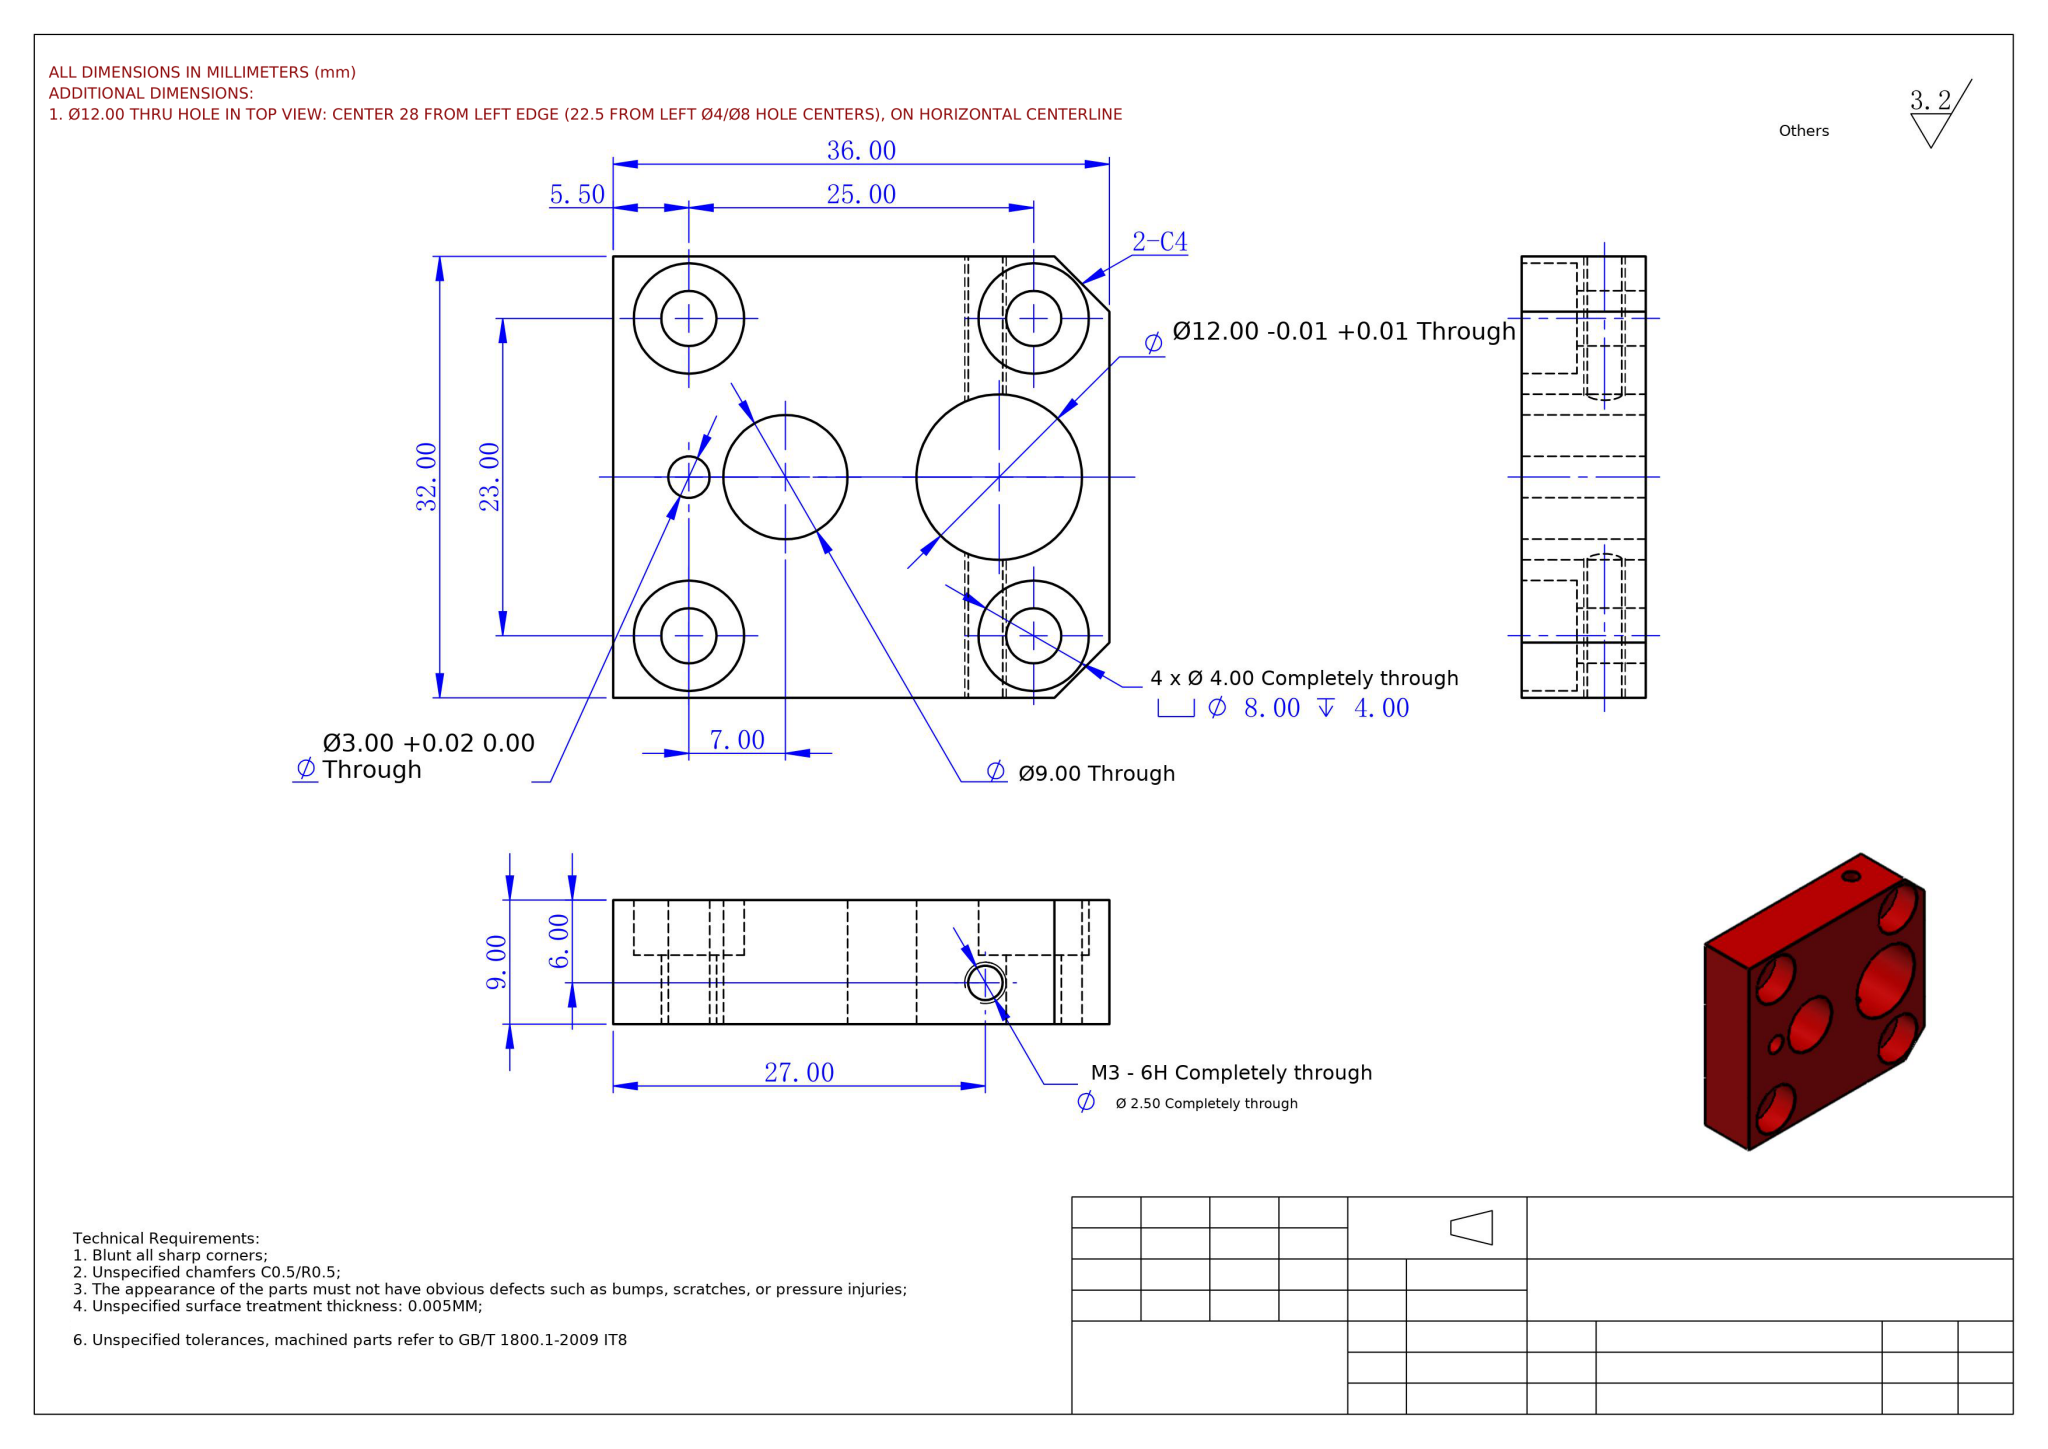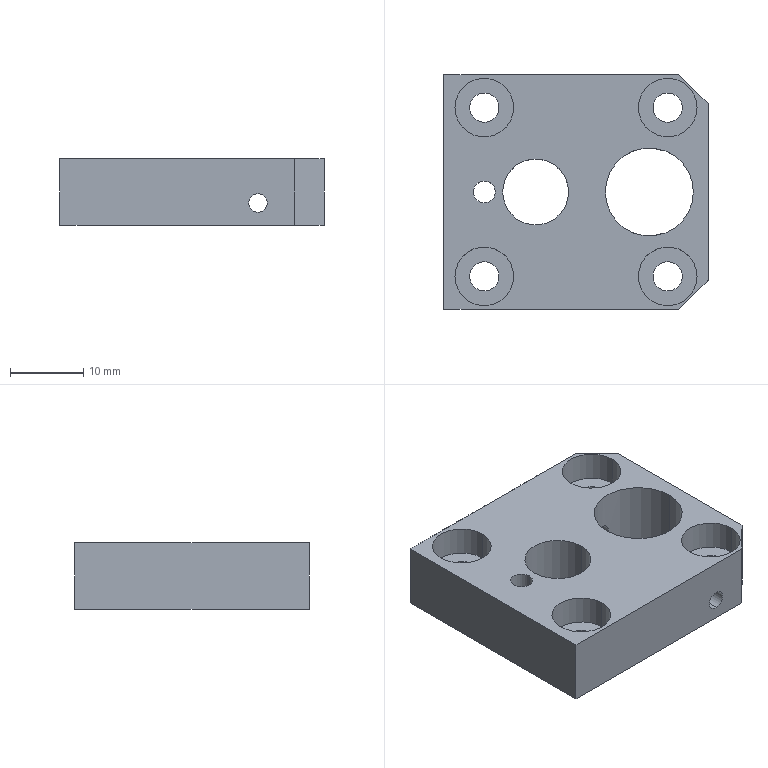Part | NX | mm | 1 solid | 38 faces | box 36 x 32 x 9 mm | volume 7415 mm3 | cylinder 26 | plane 12 | commonest cylinder face diameters 8 x8 4 x8 2.5 x4 3 x2 9 x2 12 x2